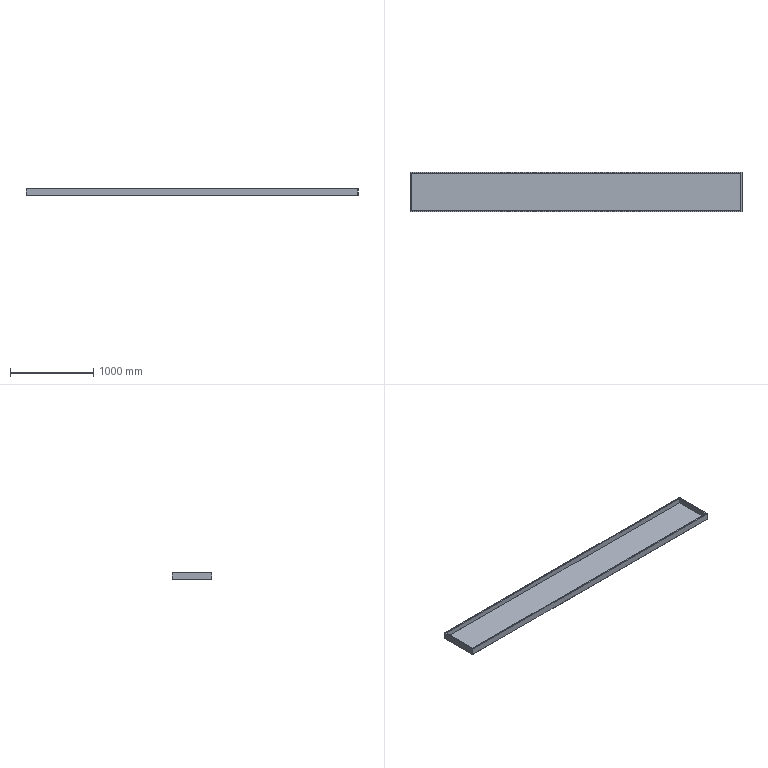Component | NX | DB6 | 1 solid | 16 faces | volume 4104477 mm3 | plane 16